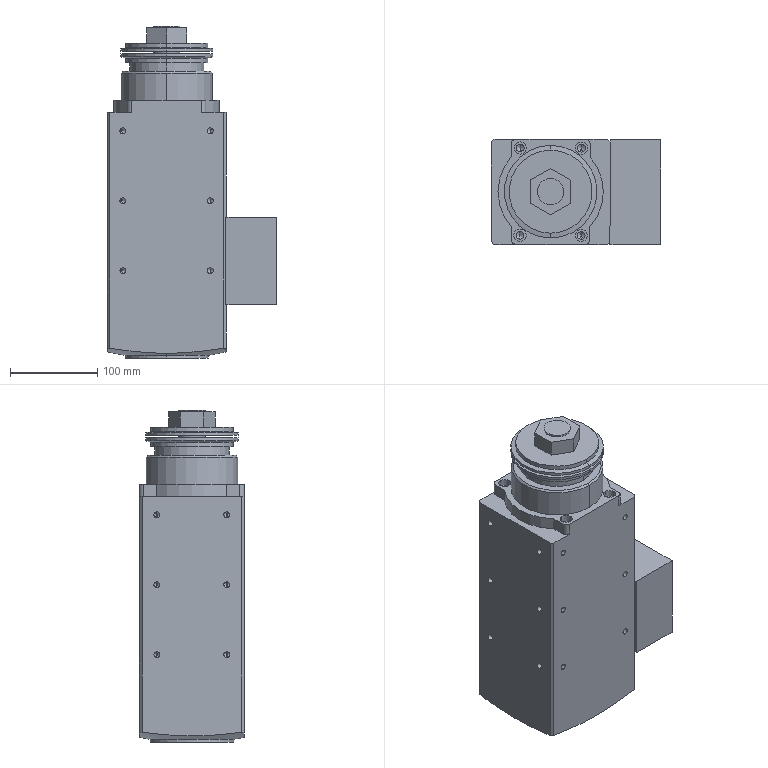Component | SolidWorks | SawingMotor-1 | 1 solid | 175 faces | box 194.24 x 120.39 x 380 mm | volume 5902858 mm3 | cylinder 76 | cone 58 | plane 41 | commonest cylinder face diameters 6.8 x36 14 x8 9 x8 95 x4 106 x4 30 x4 10 x4 105 x2
build123d program:
from build123d import *

# Parameters (mm, degrees)
BOSS_EXTRUDE1_DEPTH                             = 278
SKETCH3_R                                       = 48
BOSS_EXTRUDE2_DEPTH                             = 3
BOSS_EXTRUDE3_DEPTH                             = 14
M8_HEX_SOCKET_HEAD_CAP_SCREW_CBORE1_D           = 9
M8_HEX_SOCKET_HEAD_CAP_SCREW_CBORE1_DEPTH       = 20
M8_HEX_SOCKET_HEAD_CAP_SCREW_CBORE1_CBORE_D     = 14
M8_HEX_SOCKET_HEAD_CAP_SCREW_CBORE1_CBORE_DEPTH = 8
M8_HEX_SOCKET_HEAD_CAP_SCREW_CBORE1_TIP         = 2.704
SKETCH7_R                                       = 52.5
BOSS_EXTRUDE4_DEPTH                             = 33
CHAMFER1_SIZE                                   = 2
SKETCH8_R                                       = 15
BOSS_EXTRUDE5_DEPTH                             = 99
BOSS_EXTRUDE6_DEPTH                             = 18
M8_TAPPED_HOLE1_D                               = 6.8
M8_TAPPED_HOLE1_DEPTH                           = 15
M8_TAPPED_HOLE1_TIP                             = 2.043
SKETCH13_W                                      = 100
SKETCH13_H                                      = 58
BOSS_EXTRUDE7_DEPTH                             = 60
M8_TAPPED_HOLE2_AT_2_COUNT                      = 2
M8_TAPPED_HOLE2_AT_2_PITCH                      = 100
LPATTERN1_COUNT                                 = 3
LPATTERN1_PITCH                                 = 80


with BuildPart() as part:
    # Sketch1 → Boss-Extrude1 (new body)
    with BuildSketch(Plane.XY):
        Polygon((-60, 65), (-57, 68), (57, 68), (60, 65), (60, -65), (57, -68), (-57, -68), (-60, -65), align=None)
    extrude(amount=-BOSS_EXTRUDE1_DEPTH)

    # Sketch2 → Cut-Revolve1 (revolve, cut)
    with BuildSketch(Plane(origin=(0, 0, 0), x_dir=(0, 0, -1), z_dir=(1, 0, 0)), mode=Mode.PRIVATE) as cut_revolve1_sk:
        Polygon((278, 48), (278, 114.436), (264.523, 114.436), align=None)
    revolve(cut_revolve1_sk.sketch.rotate(Axis((0, 0, 1000), (0, 0, -1)), 90), axis=Axis((0, 0, 1000), (0, 0, -1)), mode=Mode.SUBTRACT)

    # Sketch3 → Boss-Extrude2 (add)
    with BuildSketch(Plane(origin=(0, 0, -278), x_dir=(-1, 0, 0), z_dir=(0, 0, -1))):
        Circle(SKETCH3_R)
    extrude(amount=BOSS_EXTRUDE2_DEPTH)

    # Sketch4 → Boss-Extrude3 (add)
    with BuildSketch(Plane.XY):
        with BuildLine():
            Line((-60, 40), (-60, -40))
            ThreePointArc((-60, -40), (-58.536, -43.536), (-55, -45))
            Line((-55, -45), (-40, -45))
            ThreePointArc((-40, -45), (0, -60.279), (40, -45))
            Line((40, -45), (55, -45))
            ThreePointArc((55, -45), (58.536, -43.536), (60, -40))
            Line((60, -40), (60, 40))
            ThreePointArc((60, 40), (58.536, 43.536), (55, 45))
            Line((55, 45), (40, 45))
            ThreePointArc((40, 45), (0, 60.279), (-40, 45))
            Line((-40, 45), (-55, 45))
            ThreePointArc((-55, 45), (-58.536, 43.536), (-60, 40))
        make_face()
    extrude(amount=BOSS_EXTRUDE3_DEPTH)

    # M8 Hex Socket Head Cap Screw CBORE1
    with Locations(Plane.XY.offset(14)):
        with Locations((-50, 35), (50, 35), (50, -35), (-50, -35)):
            CounterBoreHole(M8_HEX_SOCKET_HEAD_CAP_SCREW_CBORE1_D / 2, M8_HEX_SOCKET_HEAD_CAP_SCREW_CBORE1_CBORE_D / 2, M8_HEX_SOCKET_HEAD_CAP_SCREW_CBORE1_CBORE_DEPTH, depth=M8_HEX_SOCKET_HEAD_CAP_SCREW_CBORE1_DEPTH)
            with Locations((0, 0, -(M8_HEX_SOCKET_HEAD_CAP_SCREW_CBORE1_DEPTH + M8_HEX_SOCKET_HEAD_CAP_SCREW_CBORE1_TIP / 2))):  # 118° drill point
                Cone(0, M8_HEX_SOCKET_HEAD_CAP_SCREW_CBORE1_D / 2, M8_HEX_SOCKET_HEAD_CAP_SCREW_CBORE1_TIP, mode=Mode.SUBTRACT)

    # Sketch7 → Boss-Extrude4 (add)
    with BuildSketch(Plane.XY.offset(14)):
        with Locations(Location((0, 0, 0), (0, 0, 180))):
            Circle(SKETCH7_R)
    extrude(amount=BOSS_EXTRUDE4_DEPTH)

    # Chamfer1
    chamfer1_edges = [part.edges().sort_by_distance(p)[0] for p in [
        (52.5, 0, 47),
    ]]
    chamfer(chamfer1_edges, length=CHAMFER1_SIZE)

    # Sketch8 → Boss-Extrude5 (add)
    with BuildSketch(Plane.XY):
        Circle(SKETCH8_R)
    extrude(amount=BOSS_EXTRUDE5_DEPTH)

    # Sketch9 → Boss-Extrude6 (add)
    with BuildSketch(Plane.XY.offset(97)):
        Polygon((26.558, 0), (13.279, 23), (-13.279, 23), (-26.558, 0), (-13.279, -23), (13.279, -23), align=None)
    extrude(amount=-BOSS_EXTRUDE6_DEPTH)

    # Sketch10 → Revolve1 (revolve)
    with BuildSketch(Plane(origin=(0, 0, 0), x_dir=(0, 0, -1), z_dir=(1, 0, 0)), mode=Mode.PRIVATE) as revolve1_sk:
        Polygon((-70, 0), (-70, 53), (-73, 53), (-74, 47.5), (-79, 47.5), (-79, 0), align=None)
        Polygon((-67, 53), (-67, 0), (-47, 0), (-47, 42.5), (-57, 42.5), (-57, 47.5), (-62, 47.5), (-64, 53), align=None)
    revolve(revolve1_sk.sketch.rotate(Axis((0, 0, 99), (0, 0, -1)), 90), axis=Axis((0, 0, 99), (0, 0, -1)))

    # M8 Tapped Hole1
    with Locations(Plane(origin=(0, -68, 0), x_dir=(-1, 0, 0), z_dir=(0, -1, 0))):
        with Locations((40, 21), (-40, 21), (40, 101), (-40, 101), (-40, 181), (40, 181)):
            Hole(M8_TAPPED_HOLE1_D / 2, depth=M8_TAPPED_HOLE1_DEPTH)
            with Locations((0, 0, -(M8_TAPPED_HOLE1_DEPTH + M8_TAPPED_HOLE1_TIP / 2))):  # 118° drill point
                Cone(0, M8_TAPPED_HOLE1_D / 2, M8_TAPPED_HOLE1_TIP, mode=Mode.SUBTRACT)

    # Sketch13 → Boss-Extrude7 (add, symmetric)
    with BuildSketch(Plane(origin=(0, 0, 0), x_dir=(0, 0, -1), z_dir=(1, 0, 0))):
        with Locations((170, 97)):
            Rectangle(SKETCH13_W, SKETCH13_H)
    extrude(amount=BOSS_EXTRUDE7_DEPTH, both=True)

    # Sketch15 → M8 Tapped Hole2 (revolve, cut)
    with BuildSketch(Plane(origin=(-60, 50, -21), x_dir=(0, 0, 1), z_dir=(0, 1, 0))):
        Polygon((0, 0), (0, 21.793), (3.4, 19.75), (3.4, 0), align=None)
    m8_tapped_hole2 = revolve(axis=Axis((-66.35, 50, -21), (1, 0, 0)), mode=Mode.SUBTRACT)

    # M8 Tapped Hole2 at 2: M8 Tapped Hole2 ×2
    with Locations(*[(0, -i * M8_TAPPED_HOLE2_AT_2_PITCH, 0) for i in range(1, M8_TAPPED_HOLE2_AT_2_COUNT)]):
        add(m8_tapped_hole2, mode=Mode.SUBTRACT)

    # LPattern1: M8 Tapped Hole2 ×3
    with Locations(*[(0, 0, -i * LPATTERN1_PITCH) for i in range(1, LPATTERN1_COUNT)]):
        add(m8_tapped_hole2, mode=Mode.SUBTRACT)

    # LPattern1 copy 1 sketch → LPattern1 copy 1 (revolve, cut)
    with BuildSketch(Plane(origin=(-60, -50, -101), x_dir=(0, 0, 1), z_dir=(0, 1, 0))):
        Polygon((0, 0), (0, 21.793), (3.4, 19.75), (3.4, 0), align=None)
    revolve(axis=Axis((-66.35, -50, -101), (1, 0, 0)), mode=Mode.SUBTRACT)

    # LPattern1 copy 2 sketch → LPattern1 copy 2 (revolve, cut)
    with BuildSketch(Plane(origin=(-60, -50, -181), x_dir=(0, 0, 1), z_dir=(0, 1, 0))):
        Polygon((0, 0), (0, 21.793), (3.4, 19.75), (3.4, 0), align=None)
    revolve(axis=Axis((-66.35, -50, -181), (1, 0, 0)), mode=Mode.SUBTRACT)

    # Mirror1: M8 Tapped Hole2 across plane
    add(m8_tapped_hole2.mirror(Plane(origin=(0, 0, 0), x_dir=(0, 0, 1), z_dir=(1, 0, 0))), mode=Mode.SUBTRACT)

    # Mirror1 copy 1 sketch → Mirror1 copy 1 (revolve, cut)
    with BuildSketch(Plane(origin=(60, -50, -21), x_dir=(0, 0, 1), z_dir=(0, 1, 0))):
        Polygon((0, 0), (0, -21.793), (3.4, -19.75), (3.4, 0), align=None)
    revolve(axis=Axis((66.35, -50, -21), (1, 0, 0)), mode=Mode.SUBTRACT)

    # Mirror1 copy 2 sketch → Mirror1 copy 2 (revolve, cut)
    with BuildSketch(Plane(origin=(60, 50, -101), x_dir=(0, 0, 1), z_dir=(0, 1, 0))):
        Polygon((0, 0), (0, -21.793), (3.4, -19.75), (3.4, 0), align=None)
    revolve(axis=Axis((66.35, 50, -101), (1, 0, 0)), mode=Mode.SUBTRACT)

    # Mirror1 copy 3 sketch → Mirror1 copy 3 (revolve, cut)
    with BuildSketch(Plane(origin=(60, 50, -181), x_dir=(0, 0, 1), z_dir=(0, 1, 0))):
        Polygon((0, 0), (0, -21.793), (3.4, -19.75), (3.4, 0), align=None)
    revolve(axis=Axis((66.35, 50, -181), (1, 0, 0)), mode=Mode.SUBTRACT)

    # Mirror1 copy 4 sketch → Mirror1 copy 4 (revolve, cut)
    with BuildSketch(Plane(origin=(60, -50, -101), x_dir=(0, 0, 1), z_dir=(0, 1, 0))):
        Polygon((0, 0), (0, -21.793), (3.4, -19.75), (3.4, 0), align=None)
    revolve(axis=Axis((66.35, -50, -101), (1, 0, 0)), mode=Mode.SUBTRACT)

    # Mirror1 copy 5 sketch → Mirror1 copy 5 (revolve, cut)
    with BuildSketch(Plane(origin=(60, -50, -181), x_dir=(0, 0, 1), z_dir=(0, 1, 0))):
        Polygon((0, 0), (0, -21.793), (3.4, -19.75), (3.4, 0), align=None)
    revolve(axis=Axis((66.35, -50, -181), (1, 0, 0)), mode=Mode.SUBTRACT)


solid = part.part

# Placed as in the assembly
solid = solid.moved(Location((-418.028, -170.45, 1001), (0, 0, -90.118)))